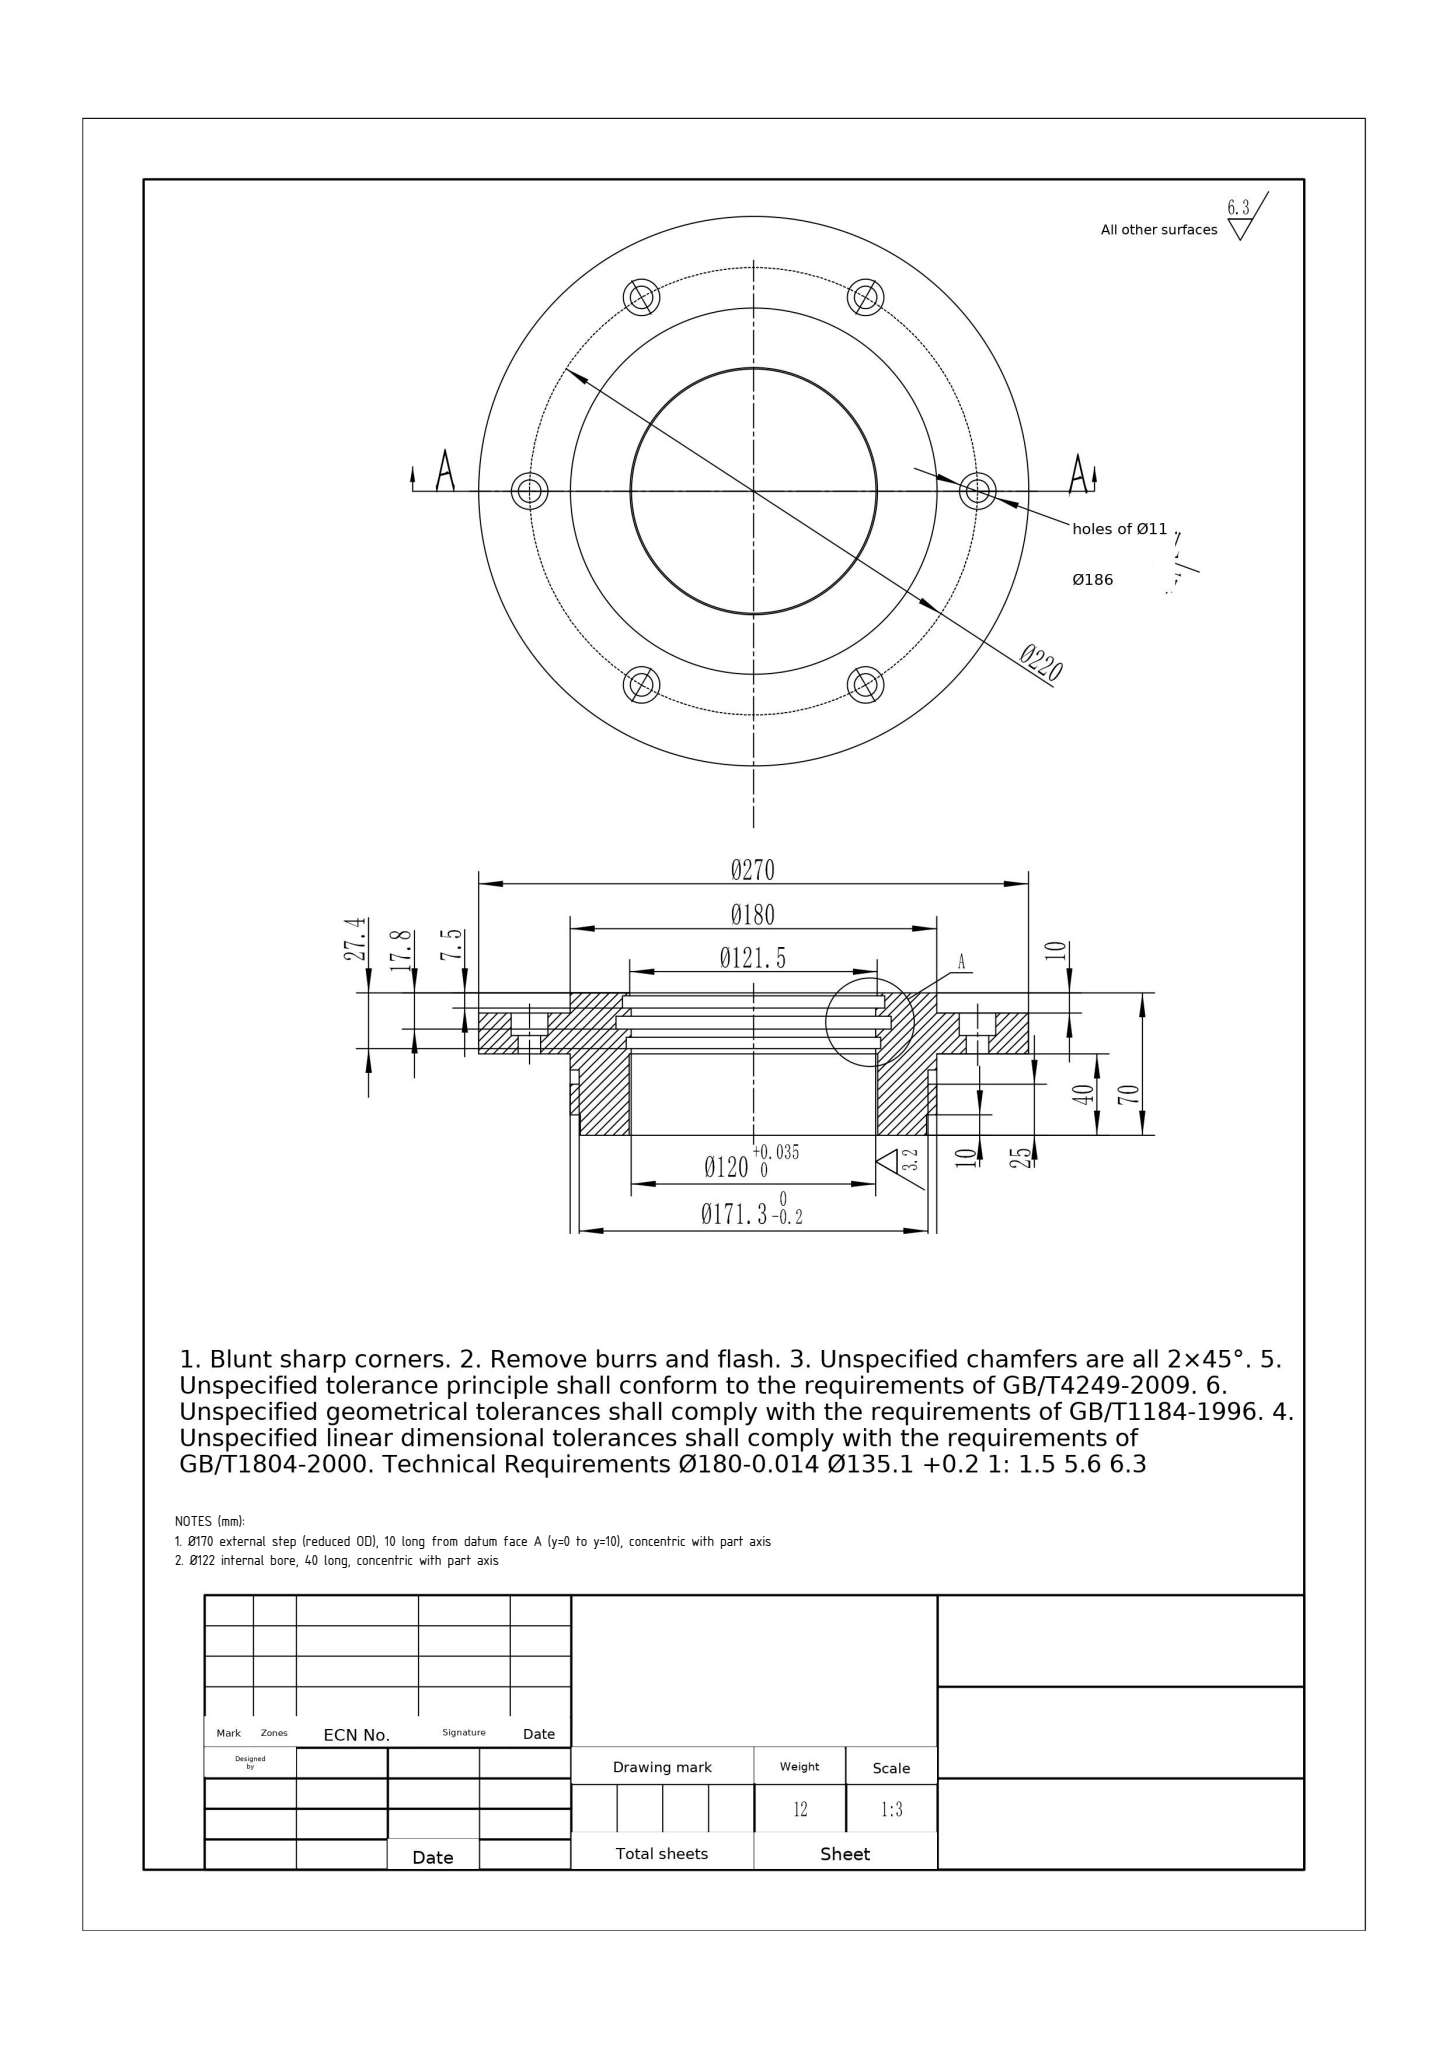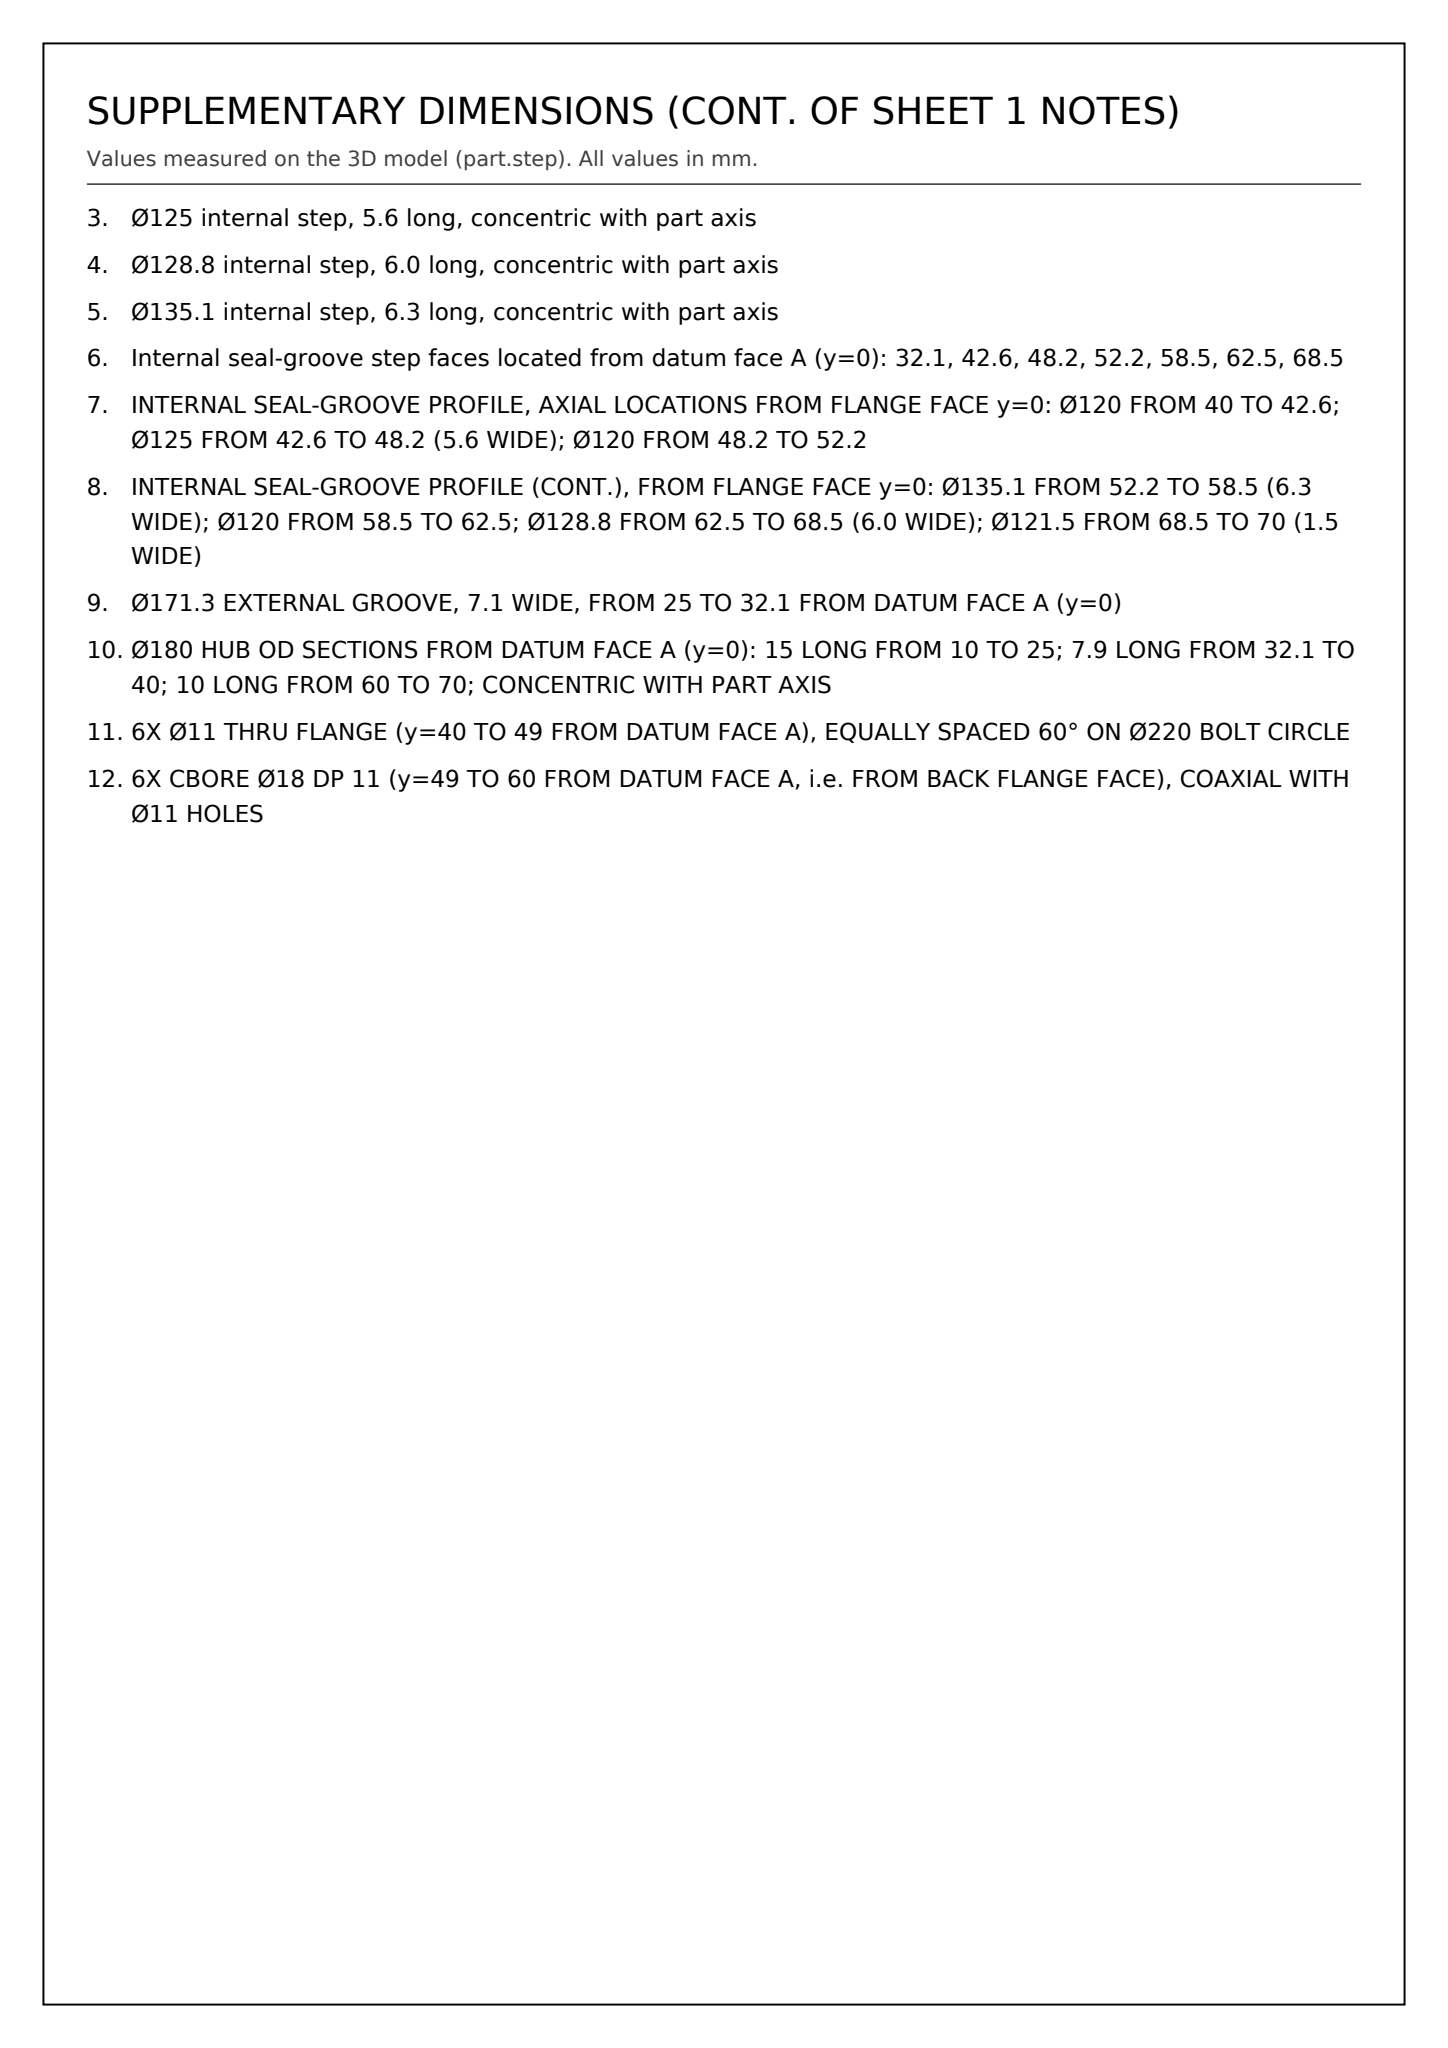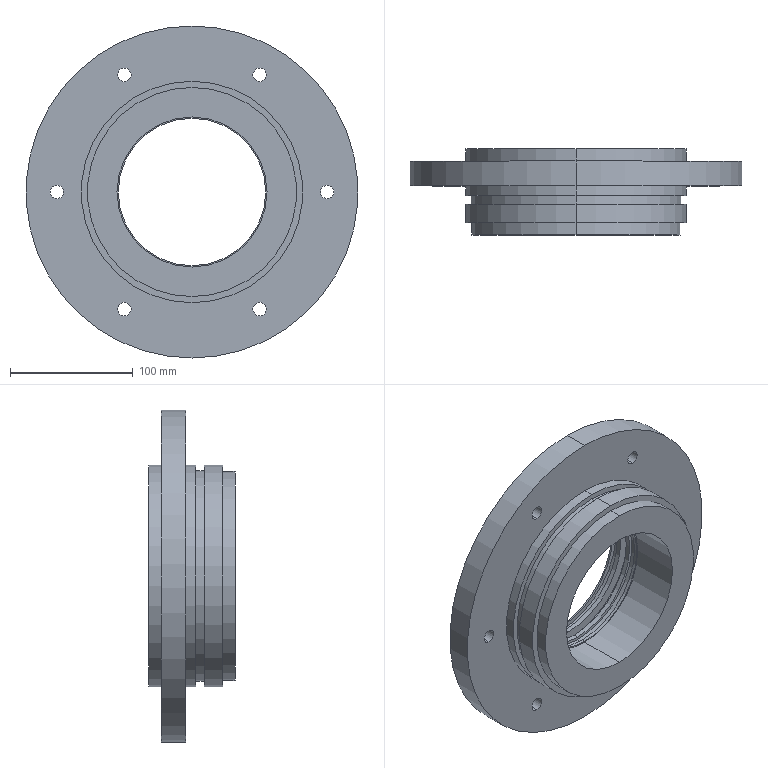Part | SolidWorks | mm | 1 solid | 72 faces | box 270 x 70 x 270 mm | volume 1508918 mm3 | cylinder 52 | plane 20 | commonest cylinder face diameters 18 x12 11 x12 180 x6 120 x6 122 x2 170 x2 171.3 x2 270 x2
Drawing notes:
Ø170 external step (reduced OD), 10 long from datum face A (y=0 to y=10), concentric with part axis | from the solid: cylinders list: ["boss/shaft", 170.0, "y", [135.0,null,135.0], from 0.0 to 10.0] - Ø170 is an external cylinder at the datum-A end, not an internal recess; no Ø170 bore exists, and the y=70 end face runs to Ø180 (extent 45..225).
Ø122 internal bore, 40 long, concentric with part axis | from the solid: cylinder [122.0,y,[135,null,135],40.0]
Ø125 internal step, 5.6 long, concentric with part axis | from the solid: cylinder [125.0,y,[135,null,135],5.6]
Ø128.8 internal step, 6.0 long, concentric with part axis | from the solid: cylinder [128.8,y,[135,null,135],6.0]
Ø135.1 internal step, 6.3 long, concentric with part axis | from the solid: cylinder [135.1,y,[135,null,135],6.3]
Internal seal-groove step faces located from datum face A (y=0): 32.1, 42.6, 48.2, 52.2, 58.5, 62.5, 68.5 | from the solid: axis_planes normal y at offsets 32.1, 42.6, 48.2, 52.2, 58.5, 62.5, 68.5
INTERNAL SEAL-GROOVE PROFILE, AXIAL LOCATIONS FROM FLANGE FACE y=0: Ø120 FROM 40 TO 42.6; Ø125 FROM 42.6 TO 48.2 (5.6 WIDE); Ø120 FROM 48.2 TO 52.2 | from the solid: cylinders Ø120 L2.6, Ø125 L5.6, Ø120 L4.0; axis planes y=40, 42.6, 48.2, 52.2
INTERNAL SEAL-GROOVE PROFILE (CONT.), FROM FLANGE FACE y=0: Ø135.1 FROM 52.2 TO 58.5 (6.3 WIDE); Ø120 FROM 58.5 TO 62.5; Ø128.8 FROM 62.5 TO 68.5 (6.0 WIDE); Ø121.5 FROM 68.5 TO 70 (1.5 WIDE) | from the solid: cylinders Ø135.1 L6.3, Ø120 L4.0, Ø128.8 L6.0, Ø121.5 L1.5; axis planes y=52.2, 58.5, 62.5, 68.5, 70
Ø171.3 EXTERNAL GROOVE, 7.1 WIDE, FROM 25 TO 32.1 FROM DATUM FACE A (y=0) | from the solid: cylinder [171.3, y, L7.1]; axis-normal planes y=25.0 and y=32.1
Ø180 HUB OD SECTIONS FROM DATUM FACE A (y=0): 15 LONG FROM 10 TO 25; 7.9 LONG FROM 32.1 TO 40; 10 LONG FROM 60 TO 70; CONCENTRIC WITH PART AXIS | from the solid: cylinders [180, y, L15], [180, y, L7.9], [180, y, L10]; axis-normal planes y=10.0, 25.0, 32.1, 40.0, 60.0, 70.0
6X Ø11 THRU FLANGE (y=40 TO 49 FROM DATUM FACE A), EQUALLY SPACED 60° ON Ø220 BOLT CIRCLE | from the solid: cylinders: six 'hole/bore' Ø11.0 axis y from 40.0 to 49.0 at (190,230.3),(190,39.7),(245,135),(25,135),(80,230.3),(80,39.7) about center (135,135) => R110 / Ø220 B.C. at 60° spacing
6X CBORE Ø18 DP 11 (y=49 TO 60 FROM DATUM FACE A, i.e. FROM BACK FLANGE FACE), COAXIAL WITH Ø11 HOLES | from the solid: cylinders: six 'hole/bore' Ø18.0 axis y from 49.0 to 60.0 at same X,Z as the Ø11 holes; axis_plane y=60.0 is the back flange face
build123d program:
from build123d import *

# Parameters (mm, degrees)
M10_HEX_SOCKET_HEAD_CAP_SCREW_CBORE1_D           = 11
M10_HEX_SOCKET_HEAD_CAP_SCREW_CBORE1_CBORE_D     = 18
M10_HEX_SOCKET_HEAD_CAP_SCREW_CBORE1_CBORE_DEPTH = 11
CIRPATTERN1_COUNT                                = 6


with BuildPart() as part:
    # Sketch1 → Revolve1 (revolve)
    with BuildSketch(Plane.XY, mode=Mode.PRIVATE) as revolve1_sk:
        Polygon((-60, 38.567), (-60, 35.967), (-61, 35.967), (-61, -4.033), (-85, -4.033), (-85, 5.967), (-90, 5.967), (-90, 20.967), (-85.65, 20.967), (-85.65, 28.067), (-90, 28.067), (-90, 35.967), (-135, 35.967), (-135, 55.967), (-90, 55.967), (-90, 65.967), (-60.75, 65.967), (-60.75, 64.467), (-64.4, 64.467), (-64.4, 58.467), (-60, 58.467), (-60, 54.467), (-67.55, 54.467), (-67.55, 48.167), (-60, 48.167), (-60, 44.167), (-62.5, 44.167), (-62.5, 38.567), align=None)
    revolve(revolve1_sk.sketch.rotate(Axis((0, 0, 0), (0, 1, 0)), 270), axis=Axis((0, 0, 0), (0, 1, 0)))

    # M10 Hex Socket Head Cap Screw CBORE1 (through all)
    with Locations(Plane(origin=(-110, 55.967, 0), x_dir=(0, 0, 1), z_dir=(0, 1, 0))):
        with Locations((0, 0)):
            m10_hex_socket_head_cap_screw_cbore1 = CounterBoreHole(M10_HEX_SOCKET_HEAD_CAP_SCREW_CBORE1_D / 2, M10_HEX_SOCKET_HEAD_CAP_SCREW_CBORE1_CBORE_D / 2, M10_HEX_SOCKET_HEAD_CAP_SCREW_CBORE1_CBORE_DEPTH)

    # CirPattern1: M10 Hex Socket Head Cap Screw CBORE1 ×6 about axis
    cirpattern1_axis = Axis((0, 0, 0), (0, 1, 0))
    for i in range(1, CIRPATTERN1_COUNT):
        add(m10_hex_socket_head_cap_screw_cbore1.rotate(cirpattern1_axis, i * 360 / CIRPATTERN1_COUNT), mode=Mode.SUBTRACT)


solid = part.part